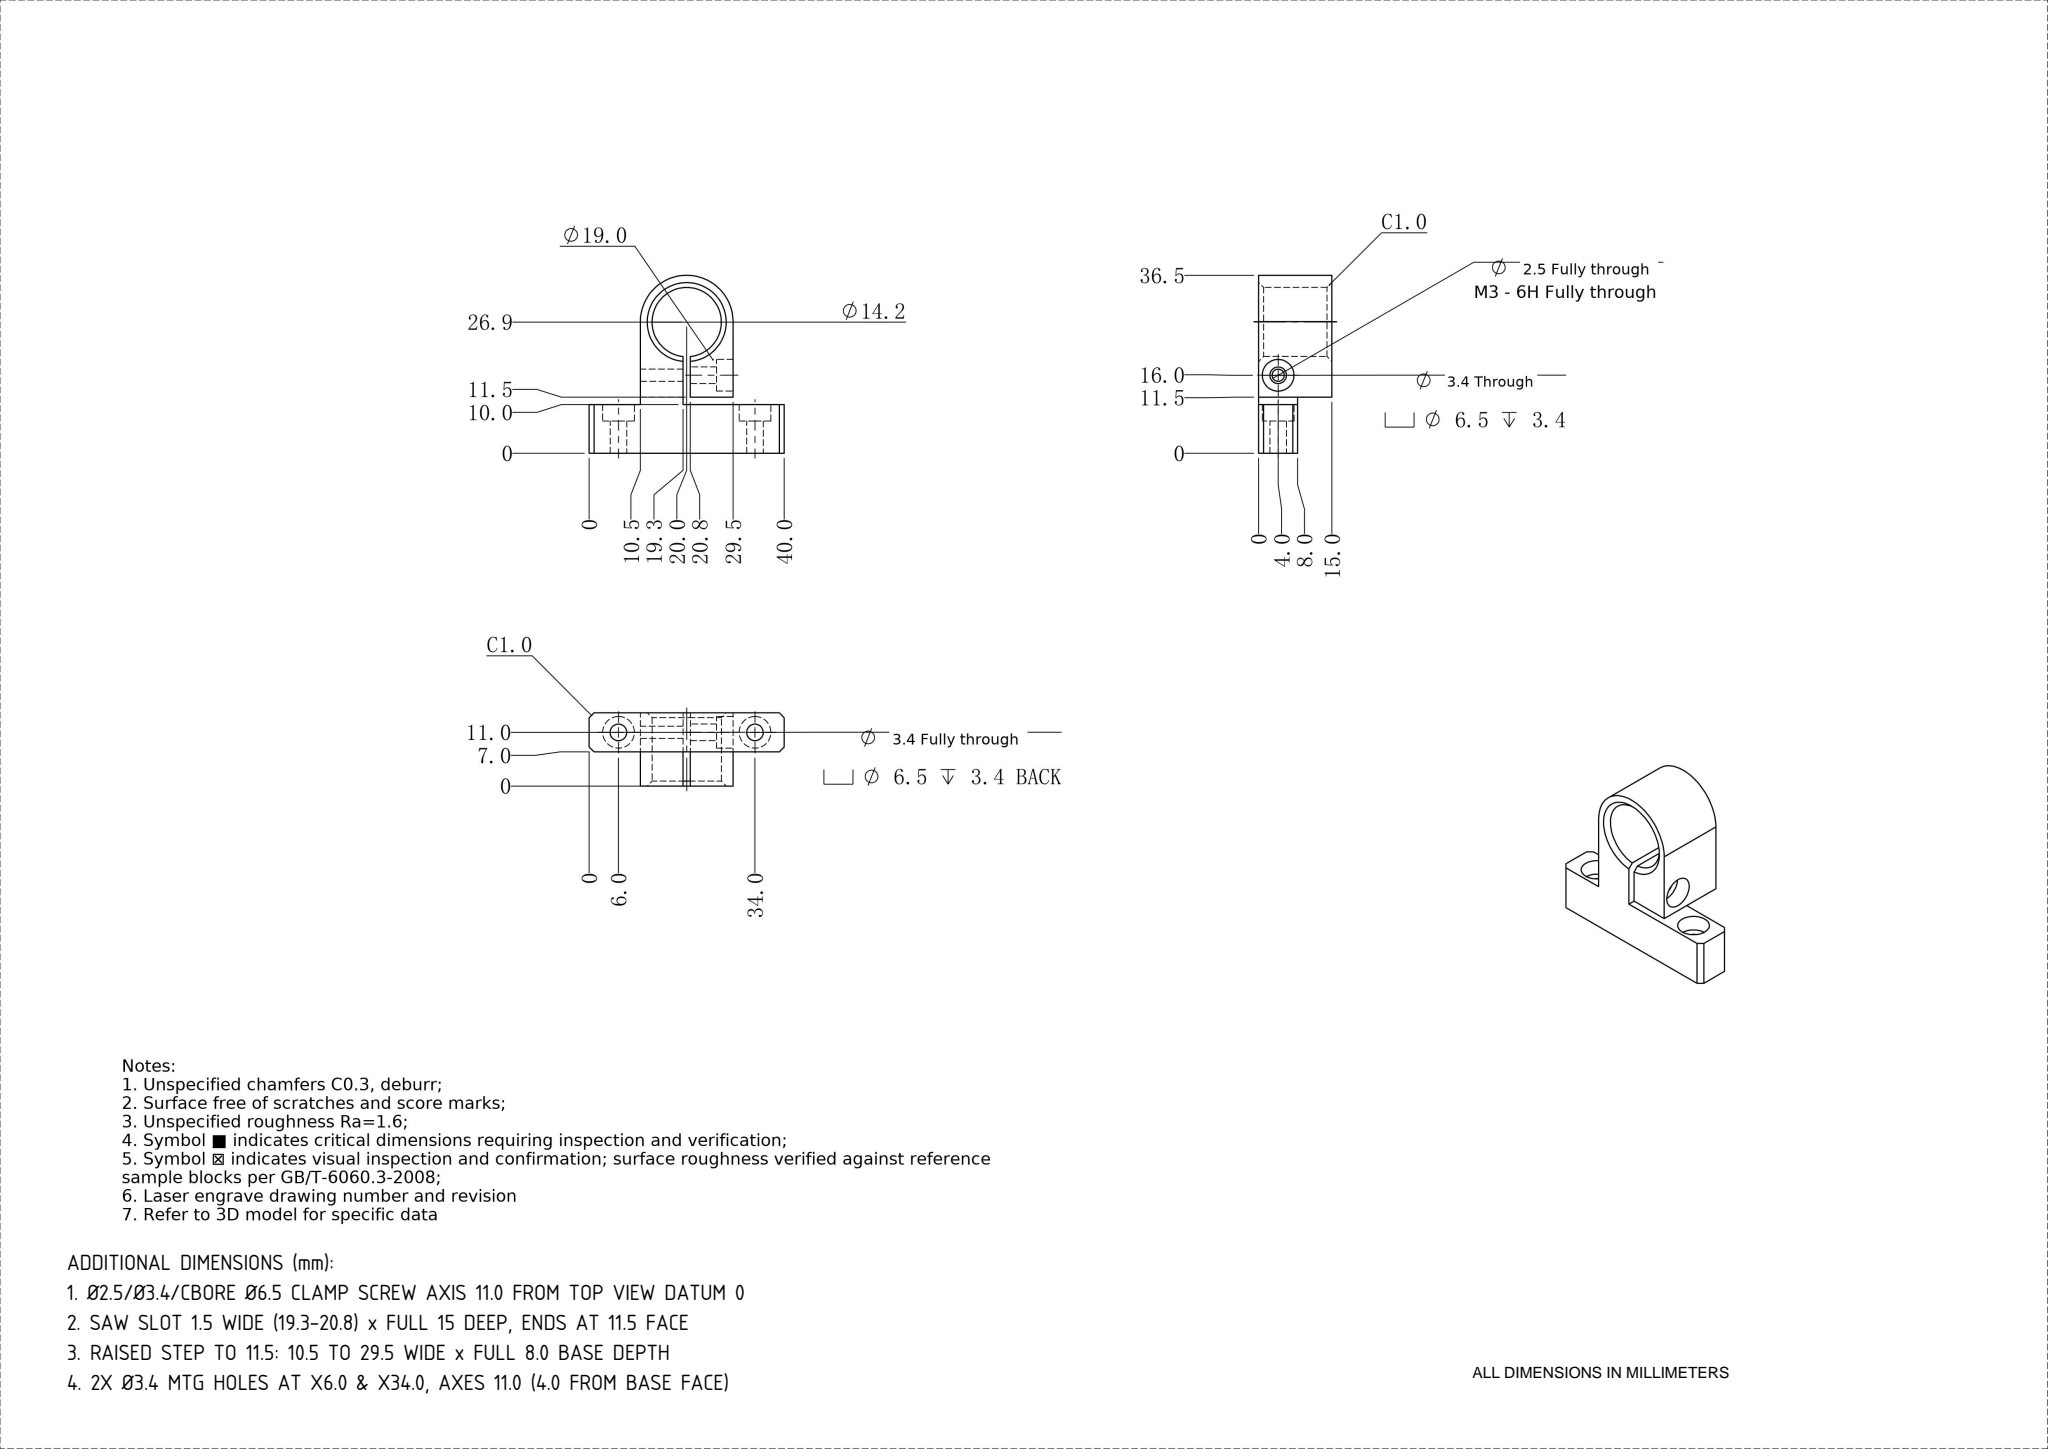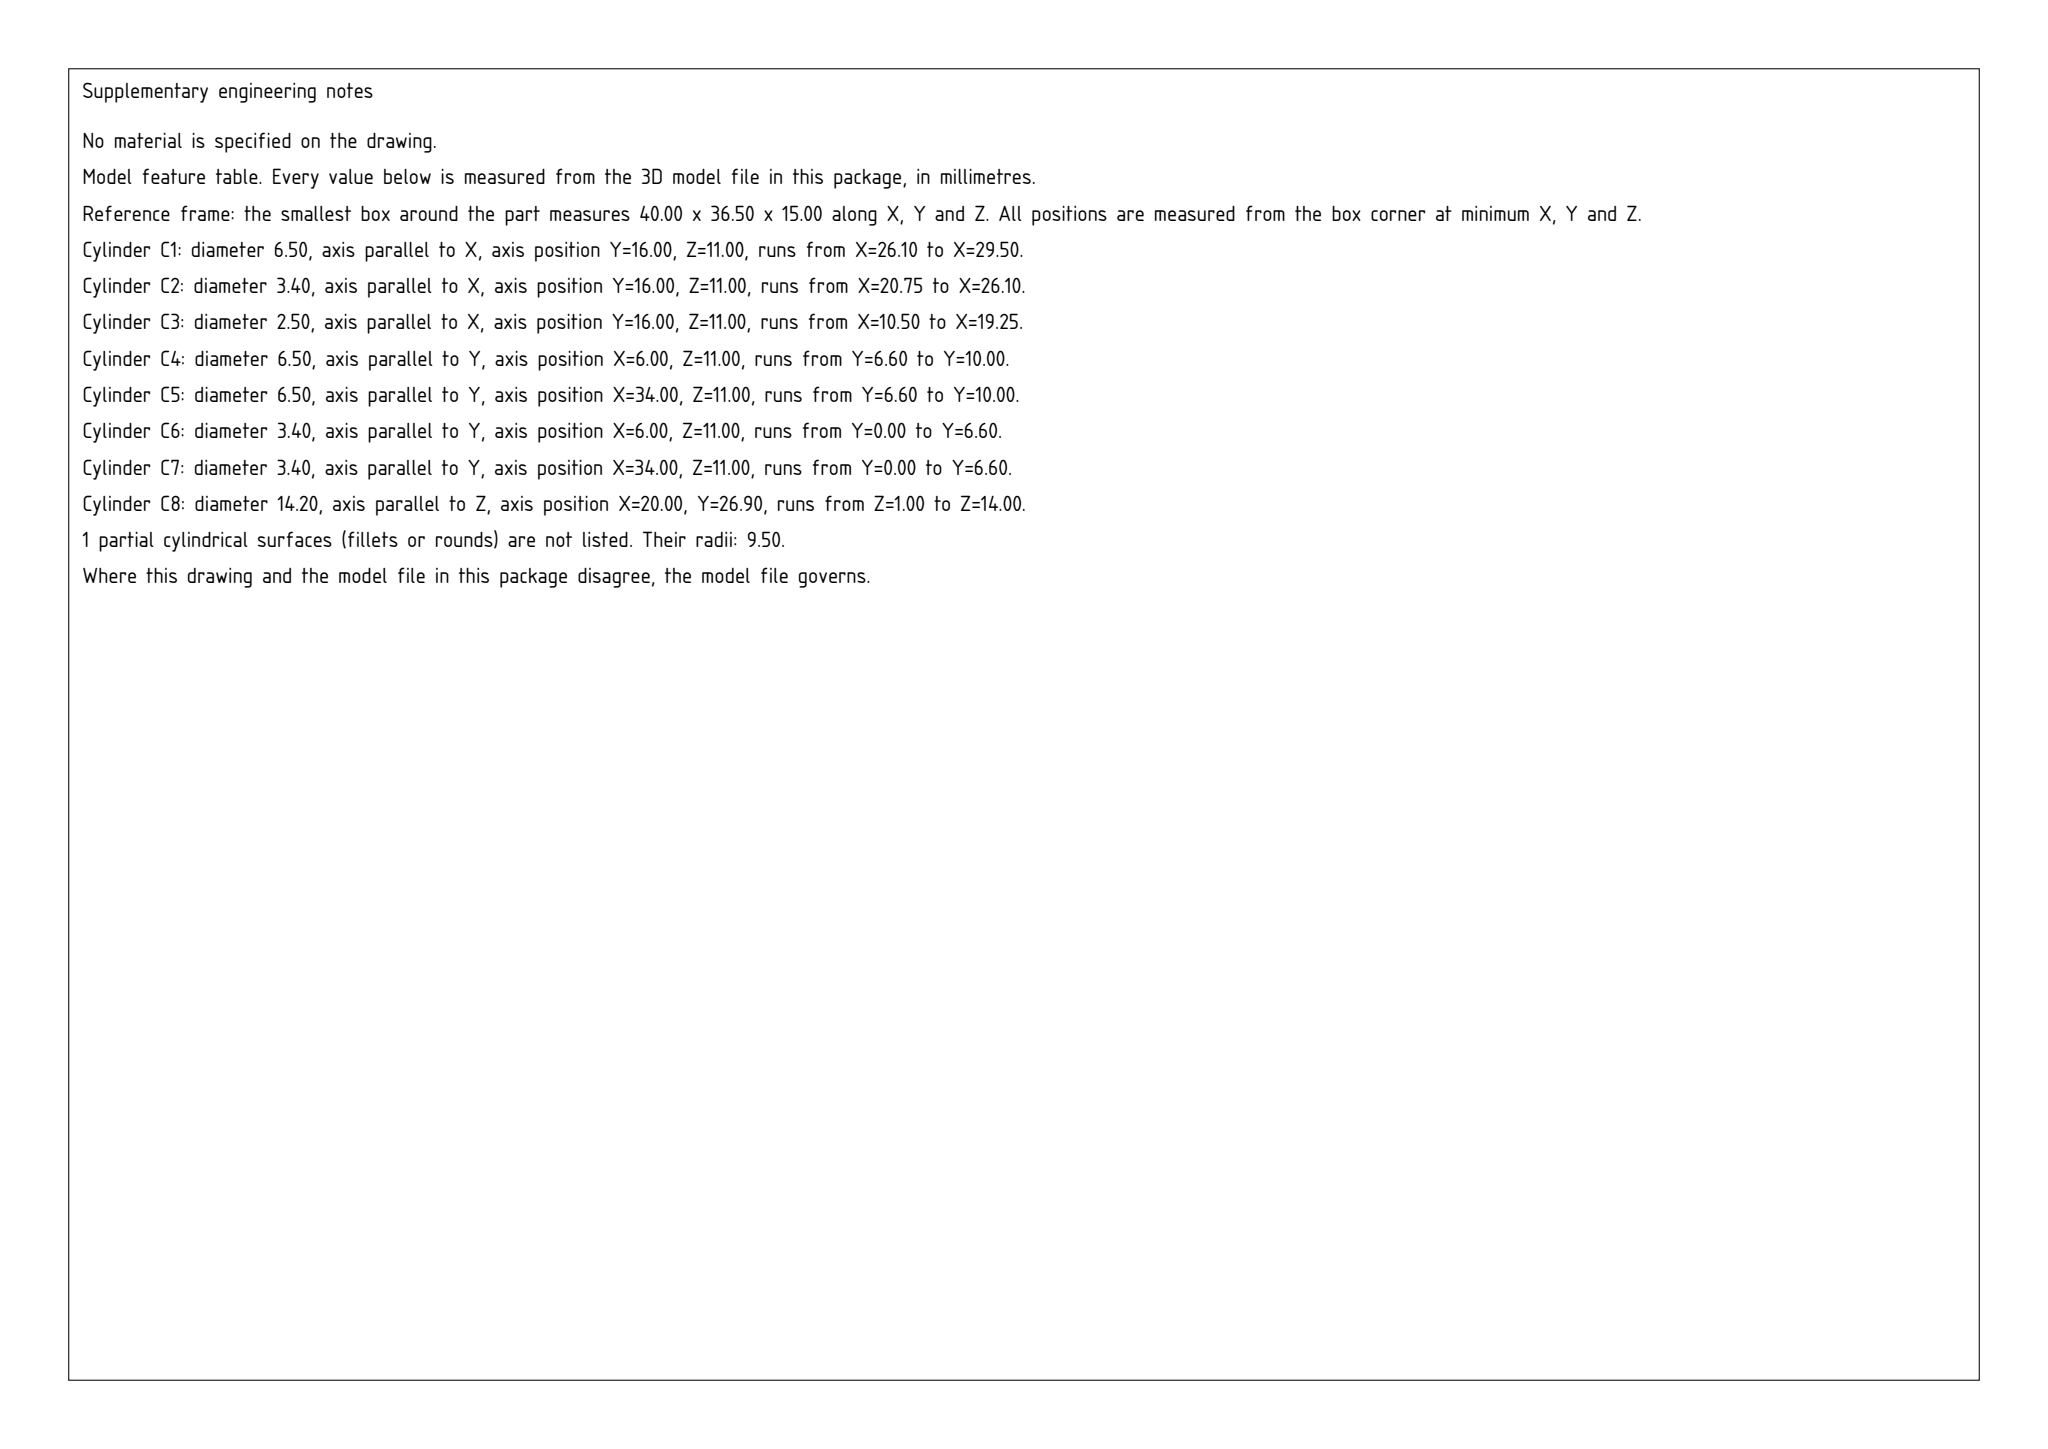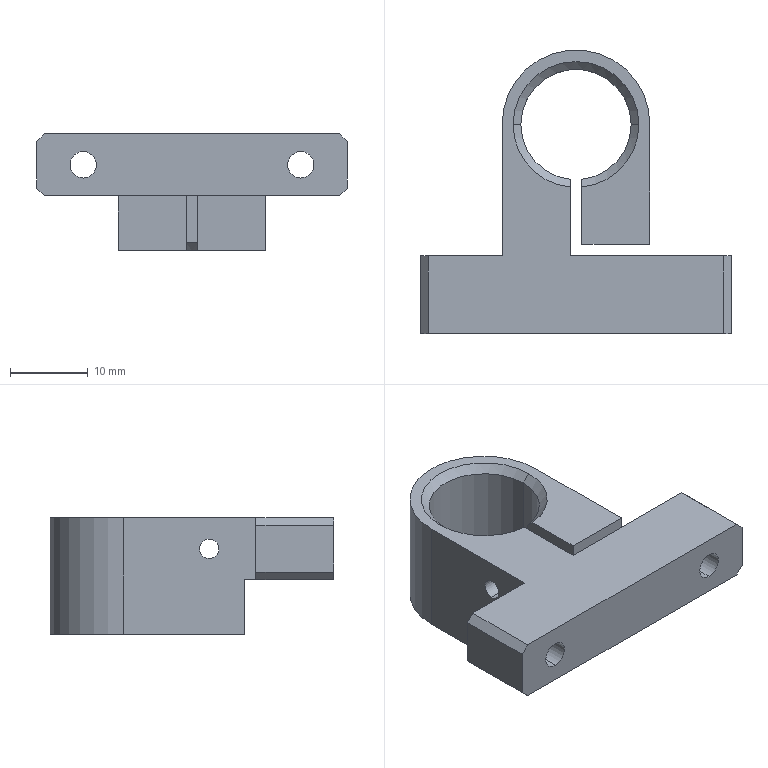Part | SolidWorks | mm | 1 solid | 45 faces | box 40 x 36.5 x 15 mm | volume 6671 mm3 | plane 21 | cylinder 18 | cone 6 | commonest cylinder face diameters 6.5 x6 3.4 x6 14.2 x3 2.5 x2 19 x1
build123d program:
from build123d import *

# Parameters (mm, degrees)
BOSS_EXTRUDE1_DEPTH                             = 15
SKETCH2_W                                       = 7
SKETCH2_H                                       = 11.5
CUT_EXTRUDE1_DEPTH                              = 29.549
SKETCH3_W                                       = 8
SKETCH3_H                                       = 10
BOSS_EXTRUDE2_DEPTH                             = 10.5
SKETCH4_W                                       = 8
SKETCH4_H                                       = 10
BOSS_EXTRUDE3_DEPTH                             = 20.75
SKETCH5_W                                       = 7.1
SKETCH5_H                                       = 15
M3_HEX_SOCKET_HEAD_CAP_SCREW_CBORE1_D           = 3.4
M3_HEX_SOCKET_HEAD_CAP_SCREW_CBORE1_CBORE_D     = 6.5
M3_HEX_SOCKET_HEAD_CAP_SCREW_CBORE1_CBORE_DEPTH = 3.4
SKETCH8_W                                       = 1.25
SKETCH8_H                                       = 19.25
M3_HEX_SOCKET_HEAD_CAP_SCREW_CBORE2_D           = 3.4
M3_HEX_SOCKET_HEAD_CAP_SCREW_CBORE2_DEPTH       = 8.75
M3_HEX_SOCKET_HEAD_CAP_SCREW_CBORE2_CBORE_D     = 6.5
M3_HEX_SOCKET_HEAD_CAP_SCREW_CBORE2_CBORE_DEPTH = 3.4
CHAMFER1_SIZE                                   = 1


with BuildPart() as part:
    # Sketch1 → Boss-Extrude1 (new body)
    with BuildSketch(Plane(origin=(0, 0, -11), x_dir=(-1, 0, 0), z_dir=(0, 0, -1))):
        with BuildLine():
            Line((-9.5, 8.75), (-9.5, -6.75))
            Line((-9.5, -6.75), (-0.75, -6.75))
            Line((-0.75, -6.75), (-0.75, 1.59))
            ThreePointArc((-0.75, 1.59), (0, 1.55), (0.75, 1.59))
            Line((0.75, 1.59), (0.75, -18.25))
            Line((0.75, -18.25), (9.5, -18.25))
            Line((9.5, -18.25), (9.5, 8.75))
            ThreePointArc((9.5, 8.75), (0, 18.25), (-9.5, 8.75))
        make_face()
    extrude(amount=-BOSS_EXTRUDE1_DEPTH)

    # Sketch2 → Cut-Extrude1 (cut, through all)
    with BuildSketch(Plane.ZY.offset(9.5)):
        with Locations((-7.5, -12.5)):
            Rectangle(SKETCH2_W, SKETCH2_H)
    extrude(amount=-CUT_EXTRUDE1_DEPTH, mode=Mode.SUBTRACT)

    # Sketch3 → Boss-Extrude2 (add)
    with BuildSketch(Plane.ZY.offset(9.5)):
        with Locations((0, -13.25)):
            Rectangle(SKETCH3_W, SKETCH3_H)
    extrude(amount=BOSS_EXTRUDE2_DEPTH)

    # Sketch4 → Boss-Extrude3 (add)
    with BuildSketch(Plane(origin=(-0.75, 0, 0), x_dir=(0, 0, -1), z_dir=(1, 0, 0))):
        with Locations((0, -13.25)):
            Rectangle(SKETCH4_W, SKETCH4_H)
    extrude(amount=BOSS_EXTRUDE3_DEPTH)

    # Sketch5 → Cut-Revolve1 (revolve, cut)
    with BuildSketch(Plane(origin=(0, 8.65, 0), x_dir=(1, 0, 0), z_dir=(0, 1, 0))):
        with Locations((3.55, 3.5)):
            Rectangle(SKETCH5_W, SKETCH5_H)
    revolve(axis=Axis((0, 8.65, -11), (0, 0, 1)), mode=Mode.SUBTRACT)

    # M3 Hex Socket Head Cap Screw CBORE1 (through all)
    with Locations(Plane(origin=(0, -8.25, 0), x_dir=(1, 0, 0), z_dir=(0, 1, 0))):
        with Locations((-14, 0), (14, 0)):
            CounterBoreHole(M3_HEX_SOCKET_HEAD_CAP_SCREW_CBORE1_D / 2, M3_HEX_SOCKET_HEAD_CAP_SCREW_CBORE1_CBORE_D / 2, M3_HEX_SOCKET_HEAD_CAP_SCREW_CBORE1_CBORE_DEPTH)

    # Sketch8 → M3 Tapped Hole1 (revolve, cut)
    with BuildSketch(Plane(origin=(-0.75, -2.25, 0), x_dir=(0, 0, -1), z_dir=(0, 1, 0))):
        with Locations((0.625, 9.625)):
            Rectangle(SKETCH8_W, SKETCH8_H)
    revolve(axis=Axis((5.6, -2.25, 0), (-1, 0, 0)), mode=Mode.SUBTRACT)

    # M3 Hex Socket Head Cap Screw CBORE2
    with Locations(Plane(origin=(9.5, 0, 0), x_dir=(0, 0, -1), z_dir=(1, 0, 0))):
        with Locations((0, -2.25)):
            CounterBoreHole(M3_HEX_SOCKET_HEAD_CAP_SCREW_CBORE2_D / 2, M3_HEX_SOCKET_HEAD_CAP_SCREW_CBORE2_CBORE_D / 2, M3_HEX_SOCKET_HEAD_CAP_SCREW_CBORE2_CBORE_DEPTH, depth=M3_HEX_SOCKET_HEAD_CAP_SCREW_CBORE2_DEPTH)

    # Chamfer1
    chamfer1_edges = [part.edges().sort_by_distance(p)[0] for p in [
        (-20, -13.25, -4),
        (-20, -13.25, 4),
        (20, -13.25, -4),
        (20, -13.25, 4),
        (0, 15.75, -11),
        (0, 15.75, 4),
    ]]
    chamfer(chamfer1_edges, length=CHAMFER1_SIZE)


solid = part.part